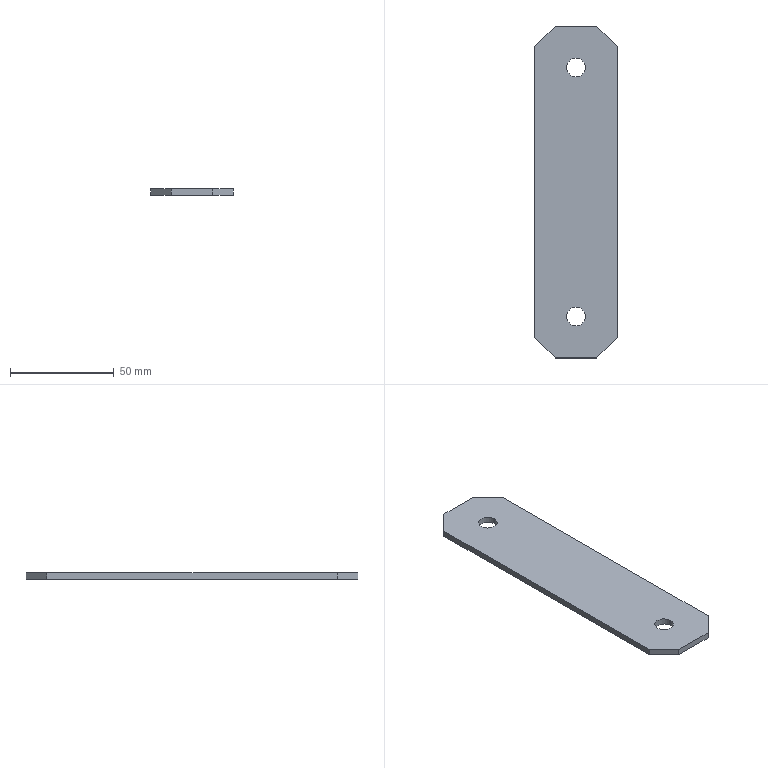Component | SolidWorks | ButtonStation-1_BracketAssembly-1_Bracket1-1 | 1 solid | 14 faces | box 40 x 160 x 3 mm | volume 18218 mm3 | plane 10 | cylinder 4 | commonest cylinder face diameters 9 x4 | material Plain Carbon Steel
STEP:
#1=COLOUR_RGB('',0.7922,0.8196,0.9333);
#2=FILL_AREA_STYLE_COLOUR('',#1);
#3=FILL_AREA_STYLE('',(#2));
#4=SURFACE_STYLE_FILL_AREA(#3);
#5=SURFACE_SIDE_STYLE('',(#4));
#6=SURFACE_STYLE_USAGE(.BOTH.,#5);
#7=PRESENTATION_STYLE_ASSIGNMENT((#6));
#8=CARTESIAN_POINT('',(6.909,20.866,16.339));
#9=VERTEX_POINT('',#8);
#10=CARTESIAN_POINT('',(7.264,20.866,16.339));
#11=VERTEX_POINT('',#10);
#12=CARTESIAN_POINT('',(7.087,20.866,16.339));
#13=DIRECTION('',(0.,0.,1.));
#14=DIRECTION('',(1.,0.,0.));
#15=AXIS2_PLACEMENT_3D('',#12,#13,#14);
#16=CIRCLE('',#15,0.1772);
#17=EDGE_CURVE('',#9,#11,#16,.T.);
#18=ORIENTED_EDGE('',*,*,#17,.F.);
#19=CARTESIAN_POINT('',(6.909,20.866,16.457));
#20=VERTEX_POINT('',#19);
#21=CARTESIAN_POINT('',(6.909,20.866,16.339));
#22=DIRECTION('',(0.,0.,1.));
#23=VECTOR('',#22,39.37);
#24=LINE('',#21,#23);
#25=EDGE_CURVE('',#9,#20,#24,.T.);
#26=ORIENTED_EDGE('',*,*,#25,.T.);
#27=CARTESIAN_POINT('',(7.264,20.866,16.457));
#28=VERTEX_POINT('',#27);
#29=CARTESIAN_POINT('',(7.087,20.866,16.457));
#30=DIRECTION('',(0.,0.,1.));
#31=DIRECTION('',(1.,0.,0.));
#32=AXIS2_PLACEMENT_3D('',#29,#30,#31);
#33=CIRCLE('',#32,0.1772);
#34=EDGE_CURVE('',#20,#28,#33,.T.);
#35=ORIENTED_EDGE('',*,*,#34,.T.);
#36=CARTESIAN_POINT('',(7.264,20.866,16.339));
#37=DIRECTION('',(0.,0.,1.));
#38=VECTOR('',#37,39.37);
#39=LINE('',#36,#38);
#40=EDGE_CURVE('',#11,#28,#39,.T.);
#41=ORIENTED_EDGE('',*,*,#40,.F.);
#42=EDGE_LOOP('',(#18,#26,#35,#41));
#43=FACE_OUTER_BOUND('',#42,.T.);
#44=CARTESIAN_POINT('',(7.087,20.866,16.339));
#45=DIRECTION('',(0.,0.,1.));
#46=DIRECTION('',(1.,0.,0.));
#47=AXIS2_PLACEMENT_3D('',#44,#45,#46);
#48=CYLINDRICAL_SURFACE('',#47,0.1772);
#49=ADVANCED_FACE('',(#43),#48,.F.);
#50=CARTESIAN_POINT('',(6.909,25.591,16.339));
#51=VERTEX_POINT('',#50);
#52=CARTESIAN_POINT('',(7.264,25.591,16.339));
#53=VERTEX_POINT('',#52);
#54=CARTESIAN_POINT('',(7.087,25.591,16.339));
#55=DIRECTION('',(0.,0.,1.));
#56=DIRECTION('',(1.,0.,0.));
#57=AXIS2_PLACEMENT_3D('',#54,#55,#56);
#58=CIRCLE('',#57,0.1772);
#59=EDGE_CURVE('',#51,#53,#58,.T.);
#60=ORIENTED_EDGE('',*,*,#59,.F.);
#61=CARTESIAN_POINT('',(6.909,25.591,16.457));
#62=VERTEX_POINT('',#61);
#63=CARTESIAN_POINT('',(6.909,25.591,16.339));
#64=DIRECTION('',(0.,0.,1.));
#65=VECTOR('',#64,39.37);
#66=LINE('',#63,#65);
#67=EDGE_CURVE('',#51,#62,#66,.T.);
#68=ORIENTED_EDGE('',*,*,#67,.T.);
#69=CARTESIAN_POINT('',(7.264,25.591,16.457));
#70=VERTEX_POINT('',#69);
#71=CARTESIAN_POINT('',(7.087,25.591,16.457));
#72=DIRECTION('',(0.,0.,1.));
#73=DIRECTION('',(1.,0.,0.));
#74=AXIS2_PLACEMENT_3D('',#71,#72,#73);
#75=CIRCLE('',#74,0.1772);
#76=EDGE_CURVE('',#62,#70,#75,.T.);
#77=ORIENTED_EDGE('',*,*,#76,.T.);
#78=CARTESIAN_POINT('',(7.264,25.591,16.339));
#79=DIRECTION('',(0.,0.,1.));
#80=VECTOR('',#79,39.37);
#81=LINE('',#78,#80);
#82=EDGE_CURVE('',#53,#70,#81,.T.);
#83=ORIENTED_EDGE('',*,*,#82,.F.);
#84=EDGE_LOOP('',(#60,#68,#77,#83));
#85=FACE_OUTER_BOUND('',#84,.T.);
#86=CARTESIAN_POINT('',(7.087,25.591,16.339));
#87=DIRECTION('',(0.,0.,1.));
#88=DIRECTION('',(1.,0.,0.));
#89=AXIS2_PLACEMENT_3D('',#86,#87,#88);
#90=CYLINDRICAL_SURFACE('',#89,0.1772);
#91=ADVANCED_FACE('',(#85),#90,.F.);
#92=CARTESIAN_POINT('',(6.299,20.472,16.457));
#93=VERTEX_POINT('',#92);
#94=CARTESIAN_POINT('',(6.299,25.984,16.457));
#95=VERTEX_POINT('',#94);
#96=CARTESIAN_POINT('',(6.299,26.378,16.457));
#97=DIRECTION('',(0.,1.,0.));
#98=VECTOR('',#97,39.37);
#99=LINE('',#96,#98);
#100=EDGE_CURVE('',#93,#95,#99,.T.);
#101=ORIENTED_EDGE('',*,*,#100,.F.);
#102=CARTESIAN_POINT('',(6.693,20.079,16.457));
#103=VERTEX_POINT('',#102);
#104=CARTESIAN_POINT('',(6.693,20.079,16.457));
#105=DIRECTION('',(-0.7071,0.7071,0.));
#106=VECTOR('',#105,39.37);
#107=LINE('',#104,#106);
#108=EDGE_CURVE('',#103,#93,#107,.T.);
#109=ORIENTED_EDGE('',*,*,#108,.F.);
#110=CARTESIAN_POINT('',(7.48,20.079,16.457));
#111=VERTEX_POINT('',#110);
#112=CARTESIAN_POINT('',(6.299,20.079,16.457));
#113=DIRECTION('',(-1.,0.,0.));
#114=VECTOR('',#113,39.37);
#115=LINE('',#112,#114);
#116=EDGE_CURVE('',#111,#103,#115,.T.);
#117=ORIENTED_EDGE('',*,*,#116,.F.);
#118=CARTESIAN_POINT('',(7.874,20.472,16.457));
#119=VERTEX_POINT('',#118);
#120=CARTESIAN_POINT('',(7.874,20.472,16.457));
#121=DIRECTION('',(-0.7071,-0.7071,0.));
#122=VECTOR('',#121,39.37);
#123=LINE('',#120,#122);
#124=EDGE_CURVE('',#119,#111,#123,.T.);
#125=ORIENTED_EDGE('',*,*,#124,.F.);
#126=CARTESIAN_POINT('',(7.874,25.984,16.457));
#127=VERTEX_POINT('',#126);
#128=CARTESIAN_POINT('',(7.874,26.378,16.457));
#129=DIRECTION('',(0.,-1.,0.));
#130=VECTOR('',#129,39.37);
#131=LINE('',#128,#130);
#132=EDGE_CURVE('',#127,#119,#131,.T.);
#133=ORIENTED_EDGE('',*,*,#132,.F.);
#134=CARTESIAN_POINT('',(7.48,26.378,16.457));
#135=VERTEX_POINT('',#134);
#136=CARTESIAN_POINT('',(7.48,26.378,16.457));
#137=DIRECTION('',(0.7071,-0.7071,0.));
#138=VECTOR('',#137,39.37);
#139=LINE('',#136,#138);
#140=EDGE_CURVE('',#135,#127,#139,.T.);
#141=ORIENTED_EDGE('',*,*,#140,.F.);
#142=CARTESIAN_POINT('',(6.693,26.378,16.457));
#143=VERTEX_POINT('',#142);
#144=CARTESIAN_POINT('',(6.299,26.378,16.457));
#145=DIRECTION('',(1.,0.,0.));
#146=VECTOR('',#145,39.37);
#147=LINE('',#144,#146);
#148=EDGE_CURVE('',#143,#135,#147,.T.);
#149=ORIENTED_EDGE('',*,*,#148,.F.);
#150=CARTESIAN_POINT('',(6.299,25.984,16.457));
#151=DIRECTION('',(0.7071,0.7071,0.));
#152=VECTOR('',#151,39.37);
#153=LINE('',#150,#152);
#154=EDGE_CURVE('',#95,#143,#153,.T.);
#155=ORIENTED_EDGE('',*,*,#154,.F.);
#156=EDGE_LOOP('',(#101,#109,#117,#125,#133,#141,#149,#155));
#157=FACE_OUTER_BOUND('',#156,.T.);
#158=CARTESIAN_POINT('',(7.087,20.866,16.457));
#159=DIRECTION('',(0.,0.,1.));
#160=DIRECTION('',(1.,0.,0.));
#161=AXIS2_PLACEMENT_3D('',#158,#159,#160);
#162=CIRCLE('',#161,0.1772);
#163=EDGE_CURVE('',#28,#20,#162,.T.);
#164=ORIENTED_EDGE('',*,*,#163,.F.);
#165=ORIENTED_EDGE('',*,*,#34,.F.);
#166=EDGE_LOOP('',(#164,#165));
#167=FACE_BOUND('',#166,.T.);
#168=CARTESIAN_POINT('',(7.087,25.591,16.457));
#169=DIRECTION('',(0.,0.,1.));
#170=DIRECTION('',(1.,0.,0.));
#171=AXIS2_PLACEMENT_3D('',#168,#169,#170);
#172=CIRCLE('',#171,0.1772);
#173=EDGE_CURVE('',#70,#62,#172,.T.);
#174=ORIENTED_EDGE('',*,*,#173,.F.);
#175=ORIENTED_EDGE('',*,*,#76,.F.);
#176=EDGE_LOOP('',(#174,#175));
#177=FACE_BOUND('',#176,.T.);
#178=CARTESIAN_POINT('',(6.299,26.378,16.457));
#179=DIRECTION('',(0.,0.,-1.));
#180=DIRECTION('',(-1.,0.,0.));
#181=AXIS2_PLACEMENT_3D('',#178,#179,#180);
#182=PLANE('',#181);
#183=ADVANCED_FACE('',(#157,#167,#177),#182,.F.);
#184=CARTESIAN_POINT('',(6.693,26.378,16.339));
#185=VERTEX_POINT('',#184);
#186=CARTESIAN_POINT('',(6.693,26.378,16.457));
#187=DIRECTION('',(0.,0.,-1.));
#188=VECTOR('',#187,39.37);
#189=LINE('',#186,#188);
#190=EDGE_CURVE('',#143,#185,#189,.T.);
#191=ORIENTED_EDGE('',*,*,#190,.T.);
#192=CARTESIAN_POINT('',(6.299,25.984,16.339));
#193=VERTEX_POINT('',#192);
#194=CARTESIAN_POINT('',(6.693,26.378,16.339));
#195=DIRECTION('',(-0.7071,-0.7071,0.));
#196=VECTOR('',#195,39.37);
#197=LINE('',#194,#196);
#198=EDGE_CURVE('',#185,#193,#197,.T.);
#199=ORIENTED_EDGE('',*,*,#198,.T.);
#200=CARTESIAN_POINT('',(6.299,25.984,16.457));
#201=DIRECTION('',(0.,0.,1.));
#202=VECTOR('',#201,39.37);
#203=LINE('',#200,#202);
#204=EDGE_CURVE('',#193,#95,#203,.T.);
#205=ORIENTED_EDGE('',*,*,#204,.T.);
#206=ORIENTED_EDGE('',*,*,#154,.T.);
#207=EDGE_LOOP('',(#191,#199,#205,#206));
#208=FACE_OUTER_BOUND('',#207,.T.);
#209=CARTESIAN_POINT('',(6.693,26.378,16.457));
#210=DIRECTION('',(-0.7071,0.7071,0.));
#211=DIRECTION('',(-0.7071,-0.7071,0.));
#212=AXIS2_PLACEMENT_3D('',#209,#210,#211);
#213=PLANE('',#212);
#214=ADVANCED_FACE('',(#208),#213,.T.);
#215=CARTESIAN_POINT('',(6.299,20.472,16.339));
#216=VERTEX_POINT('',#215);
#217=CARTESIAN_POINT('',(6.299,20.079,16.339));
#218=DIRECTION('',(0.,1.,0.));
#219=VECTOR('',#218,39.37);
#220=LINE('',#217,#219);
#221=EDGE_CURVE('',#216,#193,#220,.T.);
#222=ORIENTED_EDGE('',*,*,#221,.F.);
#223=CARTESIAN_POINT('',(6.299,20.472,16.457));
#224=DIRECTION('',(0.,0.,-1.));
#225=VECTOR('',#224,39.37);
#226=LINE('',#223,#225);
#227=EDGE_CURVE('',#93,#216,#226,.T.);
#228=ORIENTED_EDGE('',*,*,#227,.F.);
#229=ORIENTED_EDGE('',*,*,#100,.T.);
#230=ORIENTED_EDGE('',*,*,#204,.F.);
#231=EDGE_LOOP('',(#222,#228,#229,#230));
#232=FACE_OUTER_BOUND('',#231,.T.);
#233=CARTESIAN_POINT('',(6.299,20.079,16.457));
#234=DIRECTION('',(1.,0.,0.));
#235=DIRECTION('',(0.,0.,-1.));
#236=AXIS2_PLACEMENT_3D('',#233,#234,#235);
#237=PLANE('',#236);
#238=ADVANCED_FACE('',(#232),#237,.F.);
#239=ORIENTED_EDGE('',*,*,#227,.T.);
#240=CARTESIAN_POINT('',(6.693,20.079,16.339));
#241=VERTEX_POINT('',#240);
#242=CARTESIAN_POINT('',(6.693,20.079,16.339));
#243=DIRECTION('',(0.7071,-0.7071,0.));
#244=VECTOR('',#243,39.37);
#245=LINE('',#242,#244);
#246=EDGE_CURVE('',#216,#241,#245,.T.);
#247=ORIENTED_EDGE('',*,*,#246,.T.);
#248=CARTESIAN_POINT('',(6.693,20.079,16.457));
#249=DIRECTION('',(0.,0.,1.));
#250=VECTOR('',#249,39.37);
#251=LINE('',#248,#250);
#252=EDGE_CURVE('',#241,#103,#251,.T.);
#253=ORIENTED_EDGE('',*,*,#252,.T.);
#254=ORIENTED_EDGE('',*,*,#108,.T.);
#255=EDGE_LOOP('',(#239,#247,#253,#254));
#256=FACE_OUTER_BOUND('',#255,.T.);
#257=CARTESIAN_POINT('',(6.693,20.079,16.457));
#258=DIRECTION('',(-0.7071,-0.7071,0.));
#259=DIRECTION('',(0.7071,-0.7071,0.));
#260=AXIS2_PLACEMENT_3D('',#257,#258,#259);
#261=PLANE('',#260);
#262=ADVANCED_FACE('',(#256),#261,.T.);
#263=CARTESIAN_POINT('',(7.48,20.079,16.339));
#264=VERTEX_POINT('',#263);
#265=CARTESIAN_POINT('',(6.299,20.079,16.339));
#266=DIRECTION('',(-1.,0.,0.));
#267=VECTOR('',#266,39.37);
#268=LINE('',#265,#267);
#269=EDGE_CURVE('',#264,#241,#268,.T.);
#270=ORIENTED_EDGE('',*,*,#269,.F.);
#271=CARTESIAN_POINT('',(7.48,20.079,16.457));
#272=DIRECTION('',(0.,0.,-1.));
#273=VECTOR('',#272,39.37);
#274=LINE('',#271,#273);
#275=EDGE_CURVE('',#111,#264,#274,.T.);
#276=ORIENTED_EDGE('',*,*,#275,.F.);
#277=ORIENTED_EDGE('',*,*,#116,.T.);
#278=ORIENTED_EDGE('',*,*,#252,.F.);
#279=EDGE_LOOP('',(#270,#276,#277,#278));
#280=FACE_OUTER_BOUND('',#279,.T.);
#281=CARTESIAN_POINT('',(6.299,20.079,16.457));
#282=DIRECTION('',(0.,1.,0.));
#283=DIRECTION('',(0.,0.,1.));
#284=AXIS2_PLACEMENT_3D('',#281,#282,#283);
#285=PLANE('',#284);
#286=ADVANCED_FACE('',(#280),#285,.F.);
#287=ORIENTED_EDGE('',*,*,#275,.T.);
#288=CARTESIAN_POINT('',(7.874,20.472,16.339));
#289=VERTEX_POINT('',#288);
#290=CARTESIAN_POINT('',(7.874,20.472,16.339));
#291=DIRECTION('',(0.7071,0.7071,0.));
#292=VECTOR('',#291,39.37);
#293=LINE('',#290,#292);
#294=EDGE_CURVE('',#264,#289,#293,.T.);
#295=ORIENTED_EDGE('',*,*,#294,.T.);
#296=CARTESIAN_POINT('',(7.874,20.472,16.457));
#297=DIRECTION('',(0.,0.,1.));
#298=VECTOR('',#297,39.37);
#299=LINE('',#296,#298);
#300=EDGE_CURVE('',#289,#119,#299,.T.);
#301=ORIENTED_EDGE('',*,*,#300,.T.);
#302=ORIENTED_EDGE('',*,*,#124,.T.);
#303=EDGE_LOOP('',(#287,#295,#301,#302));
#304=FACE_OUTER_BOUND('',#303,.T.);
#305=CARTESIAN_POINT('',(7.874,20.472,16.457));
#306=DIRECTION('',(0.7071,-0.7071,0.));
#307=DIRECTION('',(0.7071,0.7071,0.));
#308=AXIS2_PLACEMENT_3D('',#305,#306,#307);
#309=PLANE('',#308);
#310=ADVANCED_FACE('',(#304),#309,.T.);
#311=CARTESIAN_POINT('',(7.874,25.984,16.339));
#312=VERTEX_POINT('',#311);
#313=CARTESIAN_POINT('',(7.874,20.079,16.339));
#314=DIRECTION('',(0.,-1.,0.));
#315=VECTOR('',#314,39.37);
#316=LINE('',#313,#315);
#317=EDGE_CURVE('',#312,#289,#316,.T.);
#318=ORIENTED_EDGE('',*,*,#317,.F.);
#319=CARTESIAN_POINT('',(7.874,25.984,16.457));
#320=DIRECTION('',(0.,0.,-1.));
#321=VECTOR('',#320,39.37);
#322=LINE('',#319,#321);
#323=EDGE_CURVE('',#127,#312,#322,.T.);
#324=ORIENTED_EDGE('',*,*,#323,.F.);
#325=ORIENTED_EDGE('',*,*,#132,.T.);
#326=ORIENTED_EDGE('',*,*,#300,.F.);
#327=EDGE_LOOP('',(#318,#324,#325,#326));
#328=FACE_OUTER_BOUND('',#327,.T.);
#329=CARTESIAN_POINT('',(7.874,20.079,16.457));
#330=DIRECTION('',(-1.,0.,0.));
#331=DIRECTION('',(0.,0.,1.));
#332=AXIS2_PLACEMENT_3D('',#329,#330,#331);
#333=PLANE('',#332);
#334=ADVANCED_FACE('',(#328),#333,.F.);
#335=ORIENTED_EDGE('',*,*,#323,.T.);
#336=CARTESIAN_POINT('',(7.48,26.378,16.339));
#337=VERTEX_POINT('',#336);
#338=CARTESIAN_POINT('',(7.874,25.984,16.339));
#339=DIRECTION('',(-0.7071,0.7071,0.));
#340=VECTOR('',#339,39.37);
#341=LINE('',#338,#340);
#342=EDGE_CURVE('',#312,#337,#341,.T.);
#343=ORIENTED_EDGE('',*,*,#342,.T.);
#344=CARTESIAN_POINT('',(7.48,26.378,16.457));
#345=DIRECTION('',(0.,0.,1.));
#346=VECTOR('',#345,39.37);
#347=LINE('',#344,#346);
#348=EDGE_CURVE('',#337,#135,#347,.T.);
#349=ORIENTED_EDGE('',*,*,#348,.T.);
#350=ORIENTED_EDGE('',*,*,#140,.T.);
#351=EDGE_LOOP('',(#335,#343,#349,#350));
#352=FACE_OUTER_BOUND('',#351,.T.);
#353=CARTESIAN_POINT('',(7.874,25.984,16.457));
#354=DIRECTION('',(0.7071,0.7071,0.));
#355=DIRECTION('',(-0.7071,0.7071,0.));
#356=AXIS2_PLACEMENT_3D('',#353,#354,#355);
#357=PLANE('',#356);
#358=ADVANCED_FACE('',(#352),#357,.T.);
#359=ORIENTED_EDGE('',*,*,#148,.T.);
#360=ORIENTED_EDGE('',*,*,#348,.F.);
#361=CARTESIAN_POINT('',(6.299,26.378,16.339));
#362=DIRECTION('',(1.,0.,0.));
#363=VECTOR('',#362,39.37);
#364=LINE('',#361,#363);
#365=EDGE_CURVE('',#185,#337,#364,.T.);
#366=ORIENTED_EDGE('',*,*,#365,.F.);
#367=ORIENTED_EDGE('',*,*,#190,.F.);
#368=EDGE_LOOP('',(#359,#360,#366,#367));
#369=FACE_OUTER_BOUND('',#368,.T.);
#370=CARTESIAN_POINT('',(6.299,26.378,16.457));
#371=DIRECTION('',(0.,-1.,0.));
#372=DIRECTION('',(0.,0.,-1.));
#373=AXIS2_PLACEMENT_3D('',#370,#371,#372);
#374=PLANE('',#373);
#375=ADVANCED_FACE('',(#369),#374,.F.);
#376=ORIENTED_EDGE('',*,*,#25,.F.);
#377=CARTESIAN_POINT('',(7.087,20.866,16.339));
#378=DIRECTION('',(0.,0.,1.));
#379=DIRECTION('',(1.,0.,0.));
#380=AXIS2_PLACEMENT_3D('',#377,#378,#379);
#381=CIRCLE('',#380,0.1772);
#382=EDGE_CURVE('',#11,#9,#381,.T.);
#383=ORIENTED_EDGE('',*,*,#382,.F.);
#384=ORIENTED_EDGE('',*,*,#40,.T.);
#385=ORIENTED_EDGE('',*,*,#163,.T.);
#386=EDGE_LOOP('',(#376,#383,#384,#385));
#387=FACE_OUTER_BOUND('',#386,.T.);
#388=CARTESIAN_POINT('',(7.087,20.866,16.339));
#389=DIRECTION('',(0.,0.,1.));
#390=DIRECTION('',(1.,0.,0.));
#391=AXIS2_PLACEMENT_3D('',#388,#389,#390);
#392=CYLINDRICAL_SURFACE('',#391,0.1772);
#393=ADVANCED_FACE('',(#387),#392,.F.);
#394=ORIENTED_EDGE('',*,*,#67,.F.);
#395=CARTESIAN_POINT('',(7.087,25.591,16.339));
#396=DIRECTION('',(0.,0.,1.));
#397=DIRECTION('',(1.,0.,0.));
#398=AXIS2_PLACEMENT_3D('',#395,#396,#397);
#399=CIRCLE('',#398,0.1772);
#400=EDGE_CURVE('',#53,#51,#399,.T.);
#401=ORIENTED_EDGE('',*,*,#400,.F.);
#402=ORIENTED_EDGE('',*,*,#82,.T.);
#403=ORIENTED_EDGE('',*,*,#173,.T.);
#404=EDGE_LOOP('',(#394,#401,#402,#403));
#405=FACE_OUTER_BOUND('',#404,.T.);
#406=CARTESIAN_POINT('',(7.087,25.591,16.339));
#407=DIRECTION('',(0.,0.,1.));
#408=DIRECTION('',(1.,0.,0.));
#409=AXIS2_PLACEMENT_3D('',#406,#407,#408);
#410=CYLINDRICAL_SURFACE('',#409,0.1772);
#411=ADVANCED_FACE('',(#405),#410,.F.);
#412=ORIENTED_EDGE('',*,*,#269,.T.);
#413=ORIENTED_EDGE('',*,*,#246,.F.);
#414=ORIENTED_EDGE('',*,*,#221,.T.);
#415=ORIENTED_EDGE('',*,*,#198,.F.);
#416=ORIENTED_EDGE('',*,*,#365,.T.);
#417=ORIENTED_EDGE('',*,*,#342,.F.);
#418=ORIENTED_EDGE('',*,*,#317,.T.);
#419=ORIENTED_EDGE('',*,*,#294,.F.);
#420=EDGE_LOOP('',(#412,#413,#414,#415,#416,#417,#418,#419));
#421=FACE_OUTER_BOUND('',#420,.T.);
#422=ORIENTED_EDGE('',*,*,#382,.T.);
#423=ORIENTED_EDGE('',*,*,#17,.T.);
#424=EDGE_LOOP('',(#422,#423));
#425=FACE_BOUND('',#424,.T.);
#426=ORIENTED_EDGE('',*,*,#400,.T.);
#427=ORIENTED_EDGE('',*,*,#59,.T.);
#428=EDGE_LOOP('',(#426,#427));
#429=FACE_BOUND('',#428,.T.);
#430=CARTESIAN_POINT('',(6.299,26.378,16.339));
#431=DIRECTION('',(0.,0.,-1.));
#432=DIRECTION('',(-1.,0.,0.));
#433=AXIS2_PLACEMENT_3D('',#430,#431,#432);
#434=PLANE('',#433);
#435=ADVANCED_FACE('',(#421,#425,#429),#434,.T.);
#436=CLOSED_SHELL('',(#49,#91,#183,#214,#238,#262,#286,#310,#334,#358,#375,#393,#411,#435));
#437=MANIFOLD_SOLID_BREP('',#436);
#438=STYLED_ITEM('',(#7),#437);
#439=(LENGTH_UNIT()NAMED_UNIT(*)SI_UNIT($,.METRE.));
#440=LENGTH_MEASURE_WITH_UNIT(LENGTH_MEASURE(0.0254),#439);
#441=DIMENSIONAL_EXPONENTS(1.,0.,0.,0.,0.,0.,0.);
#442=(CONVERSION_BASED_UNIT('',#440)LENGTH_UNIT()NAMED_UNIT(#441));
#443=UNCERTAINTY_MEASURE_WITH_UNIT(LENGTH_MEASURE(0.00001),#442,'','');
#444=(NAMED_UNIT(*)PLANE_ANGLE_UNIT()SI_UNIT($,.RADIAN.));
#445=(NAMED_UNIT(*)SI_UNIT($,.STERADIAN.)SOLID_ANGLE_UNIT());
#446=(GEOMETRIC_REPRESENTATION_CONTEXT(3)GLOBAL_UNCERTAINTY_ASSIGNED_CONTEXT((#443))GLOBAL_UNIT_ASSIGNED_CONTEXT((#442,#444,#445))REPRESENTATION_CONTEXT('',''));
#447=MECHANICAL_DESIGN_GEOMETRIC_PRESENTATION_REPRESENTATION('',(#438),#446);
#448=PRESENTATION_LAYER_ASSIGNMENT('','',(#438));
#449=CARTESIAN_POINT('',(0.,0.,0.));
#450=DIRECTION('',(0.,0.,1.));
#451=DIRECTION('',(1.,0.,0.));
#452=AXIS2_PLACEMENT_3D('',#449,#450,#451);
#453=(LENGTH_UNIT()NAMED_UNIT(*)SI_UNIT($,.METRE.));
#454=LENGTH_MEASURE_WITH_UNIT(LENGTH_MEASURE(0.0254),#453);
#455=DIMENSIONAL_EXPONENTS(1.,0.,0.,0.,0.,0.,0.);
#456=(CONVERSION_BASED_UNIT('',#454)LENGTH_UNIT()NAMED_UNIT(#455));
#457=UNCERTAINTY_MEASURE_WITH_UNIT(LENGTH_MEASURE(0.00001),#456,'','');
#458=(NAMED_UNIT(*)PLANE_ANGLE_UNIT()SI_UNIT($,.RADIAN.));
#459=(NAMED_UNIT(*)SI_UNIT($,.STERADIAN.)SOLID_ANGLE_UNIT());
#460=(GEOMETRIC_REPRESENTATION_CONTEXT(3)GLOBAL_UNCERTAINTY_ASSIGNED_CONTEXT((#457))GLOBAL_UNIT_ASSIGNED_CONTEXT((#456,#458,#459))REPRESENTATION_CONTEXT('',''));
#461=ADVANCED_BREP_SHAPE_REPRESENTATION('',(#437,#452),#460);